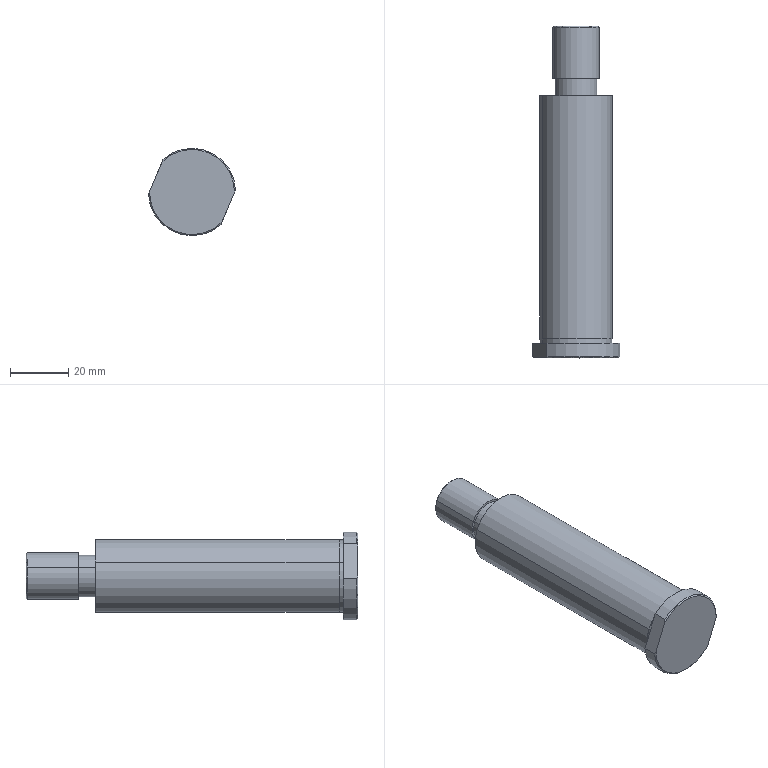Component | SolidWorks | ShaftDiameterToleranceOptionalTypeBHingePin[KPVHBH25-85]-1 | 1 solid | 22 faces | box 29.95 x 114 x 30 mm | volume 49702 mm3 | cylinder 10 | plane 8 | cone 4 | commonest cylinder face diameters 16 x2 14.4 x2 25 x2 24.8 x2 30 x2
STEP:
#1=CARTESIAN_POINT('',(4.981,-6.488,23.736));
#2=VERTEX_POINT('',#1);
#3=CARTESIAN_POINT('',(5.534,-6.488,23.508));
#4=VERTEX_POINT('',#3);
#5=CARTESIAN_POINT('',(5.257,-6.488,23.622));
#6=DIRECTION('',(-0.,1.,-0.));
#7=DIRECTION('',(0.9242,0.,-0.3818));
#8=AXIS2_PLACEMENT_3D('',#5,#6,#7);
#9=CIRCLE('',#8,0.2992);
#10=EDGE_CURVE('',#2,#4,#9,.T.);
#11=ORIENTED_EDGE('',*,*,#10,.F.);
#12=CARTESIAN_POINT('',(4.966,-6.504,23.742));
#13=VERTEX_POINT('',#12);
#14=CARTESIAN_POINT('',(4.966,-6.504,23.742));
#15=DIRECTION('',(-0.6535,-0.7071,0.27));
#16=VECTOR('',#15,39.37);
#17=LINE('',#14,#16);
#18=EDGE_CURVE('',#2,#13,#17,.T.);
#19=ORIENTED_EDGE('',*,*,#18,.T.);
#20=CARTESIAN_POINT('',(5.548,-6.504,23.502));
#21=VERTEX_POINT('',#20);
#22=CARTESIAN_POINT('',(5.257,-6.504,23.622));
#23=DIRECTION('',(0.,-1.,0.));
#24=DIRECTION('',(0.9242,0.,-0.3818));
#25=AXIS2_PLACEMENT_3D('',#22,#23,#24);
#26=CIRCLE('',#25,0.315);
#27=EDGE_CURVE('',#21,#13,#26,.T.);
#28=ORIENTED_EDGE('',*,*,#27,.F.);
#29=CARTESIAN_POINT('',(5.548,-6.504,23.502));
#30=DIRECTION('',(0.6535,-0.7071,-0.27));
#31=VECTOR('',#30,39.37);
#32=LINE('',#29,#31);
#33=EDGE_CURVE('',#4,#21,#32,.T.);
#34=ORIENTED_EDGE('',*,*,#33,.F.);
#35=EDGE_LOOP('',(#11,#19,#28,#34));
#36=FACE_OUTER_BOUND('',#35,.T.);
#37=CARTESIAN_POINT('',(5.257,-6.504,23.622));
#38=DIRECTION('',(0.,-1.,0.));
#39=DIRECTION('',(0.9242,0.,-0.3818));
#40=AXIS2_PLACEMENT_3D('',#37,#38,#39);
#41=CONICAL_SURFACE('',#40,0.315,0.7854);
#42=ADVANCED_FACE('',(#36),#41,.T.);
#43=ORIENTED_EDGE('',*,*,#27,.T.);
#44=CARTESIAN_POINT('',(4.966,-7.196,23.742));
#45=VERTEX_POINT('',#44);
#46=CARTESIAN_POINT('',(4.966,-10.976,23.742));
#47=DIRECTION('',(0.,-1.,0.));
#48=VECTOR('',#47,39.37);
#49=LINE('',#46,#48);
#50=EDGE_CURVE('',#13,#45,#49,.T.);
#51=ORIENTED_EDGE('',*,*,#50,.T.);
#52=CARTESIAN_POINT('',(5.548,-7.196,23.502));
#53=VERTEX_POINT('',#52);
#54=CARTESIAN_POINT('',(5.257,-7.196,23.622));
#55=DIRECTION('',(0.,-1.,0.));
#56=DIRECTION('',(0.9242,0.,-0.3818));
#57=AXIS2_PLACEMENT_3D('',#54,#55,#56);
#58=CIRCLE('',#57,0.315);
#59=EDGE_CURVE('',#53,#45,#58,.T.);
#60=ORIENTED_EDGE('',*,*,#59,.F.);
#61=CARTESIAN_POINT('',(5.548,-10.976,23.502));
#62=DIRECTION('',(0.,-1.,0.));
#63=VECTOR('',#62,39.37);
#64=LINE('',#61,#63);
#65=EDGE_CURVE('',#21,#53,#64,.T.);
#66=ORIENTED_EDGE('',*,*,#65,.F.);
#67=EDGE_LOOP('',(#43,#51,#60,#66));
#68=FACE_OUTER_BOUND('',#67,.T.);
#69=CARTESIAN_POINT('',(5.257,-10.976,23.622));
#70=DIRECTION('',(0.,-1.,0.));
#71=DIRECTION('',(0.9242,0.,-0.3818));
#72=AXIS2_PLACEMENT_3D('',#69,#70,#71);
#73=CYLINDRICAL_SURFACE('',#72,0.315);
#74=ADVANCED_FACE('',(#68),#73,.T.);
#75=CARTESIAN_POINT('',(5.519,-7.196,23.514));
#76=VERTEX_POINT('',#75);
#77=CARTESIAN_POINT('',(4.995,-7.196,23.73));
#78=VERTEX_POINT('',#77);
#79=CARTESIAN_POINT('',(5.257,-7.196,23.622));
#80=DIRECTION('',(0.,-1.,0.));
#81=DIRECTION('',(0.9242,0.,-0.3818));
#82=AXIS2_PLACEMENT_3D('',#79,#80,#81);
#83=CIRCLE('',#82,0.2835);
#84=EDGE_CURVE('',#76,#78,#83,.T.);
#85=ORIENTED_EDGE('',*,*,#84,.T.);
#86=CARTESIAN_POINT('',(4.995,-7.433,23.73));
#87=VERTEX_POINT('',#86);
#88=CARTESIAN_POINT('',(4.995,-10.976,23.73));
#89=DIRECTION('',(0.,-1.,0.));
#90=VECTOR('',#89,39.37);
#91=LINE('',#88,#90);
#92=EDGE_CURVE('',#78,#87,#91,.T.);
#93=ORIENTED_EDGE('',*,*,#92,.T.);
#94=CARTESIAN_POINT('',(5.519,-7.433,23.514));
#95=VERTEX_POINT('',#94);
#96=CARTESIAN_POINT('',(5.257,-7.433,23.622));
#97=DIRECTION('',(0.,-1.,0.));
#98=DIRECTION('',(0.9242,0.,-0.3818));
#99=AXIS2_PLACEMENT_3D('',#96,#97,#98);
#100=CIRCLE('',#99,0.2835);
#101=EDGE_CURVE('',#95,#87,#100,.T.);
#102=ORIENTED_EDGE('',*,*,#101,.F.);
#103=CARTESIAN_POINT('',(5.519,-10.976,23.514));
#104=DIRECTION('',(0.,-1.,0.));
#105=VECTOR('',#104,39.37);
#106=LINE('',#103,#105);
#107=EDGE_CURVE('',#76,#95,#106,.T.);
#108=ORIENTED_EDGE('',*,*,#107,.F.);
#109=EDGE_LOOP('',(#85,#93,#102,#108));
#110=FACE_OUTER_BOUND('',#109,.T.);
#111=CARTESIAN_POINT('',(5.257,-10.976,23.622));
#112=DIRECTION('',(0.,-1.,0.));
#113=DIRECTION('',(0.9242,0.,-0.3818));
#114=AXIS2_PLACEMENT_3D('',#111,#112,#113);
#115=CYLINDRICAL_SURFACE('',#114,0.2835);
#116=ADVANCED_FACE('',(#110),#115,.T.);
#117=CARTESIAN_POINT('',(5.712,-7.433,23.434));
#118=VERTEX_POINT('',#117);
#119=CARTESIAN_POINT('',(4.802,-7.433,23.81));
#120=VERTEX_POINT('',#119);
#121=CARTESIAN_POINT('',(5.257,-7.433,23.622));
#122=DIRECTION('',(0.,-1.,0.));
#123=DIRECTION('',(0.9242,0.,-0.3818));
#124=AXIS2_PLACEMENT_3D('',#121,#122,#123);
#125=CIRCLE('',#124,0.4921);
#126=EDGE_CURVE('',#118,#120,#125,.T.);
#127=ORIENTED_EDGE('',*,*,#126,.T.);
#128=CARTESIAN_POINT('',(4.802,-10.72,23.81));
#129=VERTEX_POINT('',#128);
#130=CARTESIAN_POINT('',(4.802,-10.976,23.81));
#131=DIRECTION('',(0.,-1.,0.));
#132=VECTOR('',#131,39.37);
#133=LINE('',#130,#132);
#134=EDGE_CURVE('',#120,#129,#133,.T.);
#135=ORIENTED_EDGE('',*,*,#134,.T.);
#136=CARTESIAN_POINT('',(5.712,-10.72,23.434));
#137=VERTEX_POINT('',#136);
#138=CARTESIAN_POINT('',(5.257,-10.72,23.622));
#139=DIRECTION('',(0.,-1.,0.));
#140=DIRECTION('',(0.9242,0.,-0.3818));
#141=AXIS2_PLACEMENT_3D('',#138,#139,#140);
#142=CIRCLE('',#141,0.4921);
#143=EDGE_CURVE('',#137,#129,#142,.T.);
#144=ORIENTED_EDGE('',*,*,#143,.F.);
#145=CARTESIAN_POINT('',(5.712,-10.976,23.434));
#146=DIRECTION('',(0.,-1.,0.));
#147=VECTOR('',#146,39.37);
#148=LINE('',#145,#147);
#149=EDGE_CURVE('',#118,#137,#148,.T.);
#150=ORIENTED_EDGE('',*,*,#149,.F.);
#151=EDGE_LOOP('',(#127,#135,#144,#150));
#152=FACE_OUTER_BOUND('',#151,.T.);
#153=CARTESIAN_POINT('',(5.257,-10.976,23.622));
#154=DIRECTION('',(0.,-1.,0.));
#155=DIRECTION('',(0.9242,0.,-0.3818));
#156=AXIS2_PLACEMENT_3D('',#153,#154,#155);
#157=CYLINDRICAL_SURFACE('',#156,0.4921);
#158=ADVANCED_FACE('',(#152),#157,.T.);
#159=CARTESIAN_POINT('',(5.708,-10.72,23.436));
#160=VERTEX_POINT('',#159);
#161=CARTESIAN_POINT('',(4.806,-10.72,23.808));
#162=VERTEX_POINT('',#161);
#163=CARTESIAN_POINT('',(5.257,-10.72,23.622));
#164=DIRECTION('',(0.,-1.,0.));
#165=DIRECTION('',(0.9242,0.,-0.3818));
#166=AXIS2_PLACEMENT_3D('',#163,#164,#165);
#167=CIRCLE('',#166,0.4882);
#168=EDGE_CURVE('',#160,#162,#167,.T.);
#169=ORIENTED_EDGE('',*,*,#168,.T.);
#170=CARTESIAN_POINT('',(4.806,-10.779,23.808));
#171=VERTEX_POINT('',#170);
#172=CARTESIAN_POINT('',(4.806,-10.976,23.808));
#173=DIRECTION('',(0.,-1.,0.));
#174=VECTOR('',#173,39.37);
#175=LINE('',#172,#174);
#176=EDGE_CURVE('',#162,#171,#175,.T.);
#177=ORIENTED_EDGE('',*,*,#176,.T.);
#178=CARTESIAN_POINT('',(5.708,-10.779,23.436));
#179=VERTEX_POINT('',#178);
#180=CARTESIAN_POINT('',(5.257,-10.779,23.622));
#181=DIRECTION('',(0.,-1.,0.));
#182=DIRECTION('',(0.9242,0.,-0.3818));
#183=AXIS2_PLACEMENT_3D('',#180,#181,#182);
#184=CIRCLE('',#183,0.4882);
#185=EDGE_CURVE('',#179,#171,#184,.T.);
#186=ORIENTED_EDGE('',*,*,#185,.F.);
#187=CARTESIAN_POINT('',(5.708,-10.976,23.436));
#188=DIRECTION('',(0.,-1.,0.));
#189=VECTOR('',#188,39.37);
#190=LINE('',#187,#189);
#191=EDGE_CURVE('',#160,#179,#190,.T.);
#192=ORIENTED_EDGE('',*,*,#191,.F.);
#193=EDGE_LOOP('',(#169,#177,#186,#192));
#194=FACE_OUTER_BOUND('',#193,.T.);
#195=CARTESIAN_POINT('',(5.257,-10.976,23.622));
#196=DIRECTION('',(0.,-1.,0.));
#197=DIRECTION('',(0.9242,0.,-0.3818));
#198=AXIS2_PLACEMENT_3D('',#195,#196,#197);
#199=CYLINDRICAL_SURFACE('',#198,0.4882);
#200=ADVANCED_FACE('',(#194),#199,.T.);
#201=CARTESIAN_POINT('',(5.65,-10.779,23.181));
#202=VERTEX_POINT('',#201);
#203=CARTESIAN_POINT('',(5.65,-10.96,23.181));
#204=VERTEX_POINT('',#203);
#205=CARTESIAN_POINT('',(5.65,-10.779,23.181));
#206=DIRECTION('',(0.,-1.,0.));
#207=VECTOR('',#206,39.37);
#208=LINE('',#205,#207);
#209=EDGE_CURVE('',#202,#204,#208,.T.);
#210=ORIENTED_EDGE('',*,*,#209,.T.);
#211=CARTESIAN_POINT('',(4.668,-10.96,23.587));
#212=VERTEX_POINT('',#211);
#213=CARTESIAN_POINT('',(5.257,-10.96,23.622));
#214=DIRECTION('',(-0.,1.,-0.));
#215=DIRECTION('',(-0.9242,-0.,0.3818));
#216=AXIS2_PLACEMENT_3D('',#213,#214,#215);
#217=CIRCLE('',#216,0.5906);
#218=EDGE_CURVE('',#204,#212,#217,.T.);
#219=ORIENTED_EDGE('',*,*,#218,.T.);
#220=CARTESIAN_POINT('',(4.668,-10.779,23.587));
#221=VERTEX_POINT('',#220);
#222=CARTESIAN_POINT('',(4.668,-10.779,23.587));
#223=DIRECTION('',(0.,-1.,0.));
#224=VECTOR('',#223,39.37);
#225=LINE('',#222,#224);
#226=EDGE_CURVE('',#221,#212,#225,.T.);
#227=ORIENTED_EDGE('',*,*,#226,.F.);
#228=CARTESIAN_POINT('',(5.257,-10.779,23.622));
#229=DIRECTION('',(0.,-1.,0.));
#230=DIRECTION('',(0.9242,0.,-0.3818));
#231=AXIS2_PLACEMENT_3D('',#228,#229,#230);
#232=CIRCLE('',#231,0.5906);
#233=EDGE_CURVE('',#221,#202,#232,.T.);
#234=ORIENTED_EDGE('',*,*,#233,.T.);
#235=EDGE_LOOP('',(#210,#219,#227,#234));
#236=FACE_OUTER_BOUND('',#235,.T.);
#237=CARTESIAN_POINT('',(5.257,-10.976,23.622));
#238=DIRECTION('',(0.,-1.,0.));
#239=DIRECTION('',(0.9242,0.,-0.3818));
#240=AXIS2_PLACEMENT_3D('',#237,#238,#239);
#241=CYLINDRICAL_SURFACE('',#240,0.5906);
#242=ADVANCED_FACE('',(#236),#241,.T.);
#243=CARTESIAN_POINT('',(4.864,-10.779,24.063));
#244=VERTEX_POINT('',#243);
#245=CARTESIAN_POINT('',(4.864,-10.96,24.063));
#246=VERTEX_POINT('',#245);
#247=CARTESIAN_POINT('',(4.864,-10.779,24.063));
#248=DIRECTION('',(0.,-1.,0.));
#249=VECTOR('',#248,39.37);
#250=LINE('',#247,#249);
#251=EDGE_CURVE('',#244,#246,#250,.T.);
#252=ORIENTED_EDGE('',*,*,#251,.T.);
#253=CARTESIAN_POINT('',(5.847,-10.96,23.657));
#254=VERTEX_POINT('',#253);
#255=CARTESIAN_POINT('',(5.257,-10.96,23.622));
#256=DIRECTION('',(-0.,1.,-0.));
#257=DIRECTION('',(-0.9242,-0.,0.3818));
#258=AXIS2_PLACEMENT_3D('',#255,#256,#257);
#259=CIRCLE('',#258,0.5906);
#260=EDGE_CURVE('',#246,#254,#259,.T.);
#261=ORIENTED_EDGE('',*,*,#260,.T.);
#262=CARTESIAN_POINT('',(5.847,-10.779,23.657));
#263=VERTEX_POINT('',#262);
#264=CARTESIAN_POINT('',(5.847,-10.779,23.657));
#265=DIRECTION('',(0.,-1.,0.));
#266=VECTOR('',#265,39.37);
#267=LINE('',#264,#266);
#268=EDGE_CURVE('',#263,#254,#267,.T.);
#269=ORIENTED_EDGE('',*,*,#268,.F.);
#270=CARTESIAN_POINT('',(5.257,-10.779,23.622));
#271=DIRECTION('',(0.,-1.,0.));
#272=DIRECTION('',(0.9242,0.,-0.3818));
#273=AXIS2_PLACEMENT_3D('',#270,#271,#272);
#274=CIRCLE('',#273,0.5906);
#275=EDGE_CURVE('',#263,#244,#274,.T.);
#276=ORIENTED_EDGE('',*,*,#275,.T.);
#277=EDGE_LOOP('',(#252,#261,#269,#276));
#278=FACE_OUTER_BOUND('',#277,.T.);
#279=CARTESIAN_POINT('',(5.257,-10.976,23.622));
#280=DIRECTION('',(0.,-1.,0.));
#281=DIRECTION('',(0.9242,0.,-0.3818));
#282=AXIS2_PLACEMENT_3D('',#279,#280,#281);
#283=CYLINDRICAL_SURFACE('',#282,0.5906);
#284=ADVANCED_FACE('',(#278),#283,.T.);
#285=ORIENTED_EDGE('',*,*,#275,.F.);
#286=CARTESIAN_POINT('',(5.847,-10.779,23.657));
#287=DIRECTION('',(-0.3818,-0.,-0.9242));
#288=VECTOR('',#287,39.37);
#289=LINE('',#286,#288);
#290=EDGE_CURVE('',#263,#202,#289,.T.);
#291=ORIENTED_EDGE('',*,*,#290,.T.);
#292=ORIENTED_EDGE('',*,*,#233,.F.);
#293=CARTESIAN_POINT('',(4.864,-10.779,24.063));
#294=DIRECTION('',(0.3818,0.,0.9242));
#295=VECTOR('',#294,39.37);
#296=LINE('',#293,#295);
#297=EDGE_CURVE('',#221,#244,#296,.T.);
#298=ORIENTED_EDGE('',*,*,#297,.T.);
#299=EDGE_LOOP('',(#285,#291,#292,#298));
#300=FACE_OUTER_BOUND('',#299,.T.);
#301=ORIENTED_EDGE('',*,*,#185,.T.);
#302=CARTESIAN_POINT('',(5.257,-10.779,23.622));
#303=DIRECTION('',(0.,-1.,0.));
#304=DIRECTION('',(0.9242,0.,-0.3818));
#305=AXIS2_PLACEMENT_3D('',#302,#303,#304);
#306=CIRCLE('',#305,0.4882);
#307=EDGE_CURVE('',#171,#179,#306,.T.);
#308=ORIENTED_EDGE('',*,*,#307,.T.);
#309=EDGE_LOOP('',(#301,#308));
#310=FACE_BOUND('',#309,.T.);
#311=CARTESIAN_POINT('',(5.483,-10.779,24.168));
#312=DIRECTION('',(0.,-1.,0.));
#313=DIRECTION('',(0.9242,0.,-0.3818));
#314=AXIS2_PLACEMENT_3D('',#311,#312,#313);
#315=PLANE('',#314);
#316=ADVANCED_FACE('',(#300,#310),#315,.F.);
#317=ORIENTED_EDGE('',*,*,#176,.F.);
#318=CARTESIAN_POINT('',(5.257,-10.72,23.622));
#319=DIRECTION('',(0.,-1.,0.));
#320=DIRECTION('',(0.9242,0.,-0.3818));
#321=AXIS2_PLACEMENT_3D('',#318,#319,#320);
#322=CIRCLE('',#321,0.4882);
#323=EDGE_CURVE('',#162,#160,#322,.T.);
#324=ORIENTED_EDGE('',*,*,#323,.T.);
#325=ORIENTED_EDGE('',*,*,#191,.T.);
#326=ORIENTED_EDGE('',*,*,#307,.F.);
#327=EDGE_LOOP('',(#317,#324,#325,#326));
#328=FACE_OUTER_BOUND('',#327,.T.);
#329=CARTESIAN_POINT('',(5.257,-10.976,23.622));
#330=DIRECTION('',(0.,-1.,0.));
#331=DIRECTION('',(0.9242,0.,-0.3818));
#332=AXIS2_PLACEMENT_3D('',#329,#330,#331);
#333=CYLINDRICAL_SURFACE('',#332,0.4882);
#334=ADVANCED_FACE('',(#328),#333,.T.);
#335=ORIENTED_EDGE('',*,*,#168,.F.);
#336=ORIENTED_EDGE('',*,*,#323,.F.);
#337=EDGE_LOOP('',(#335,#336));
#338=FACE_BOUND('',#337,.T.);
#339=ORIENTED_EDGE('',*,*,#143,.T.);
#340=CARTESIAN_POINT('',(5.257,-10.72,23.622));
#341=DIRECTION('',(0.,-1.,0.));
#342=DIRECTION('',(0.9242,0.,-0.3818));
#343=AXIS2_PLACEMENT_3D('',#340,#341,#342);
#344=CIRCLE('',#343,0.4921);
#345=EDGE_CURVE('',#129,#137,#344,.T.);
#346=ORIENTED_EDGE('',*,*,#345,.T.);
#347=EDGE_LOOP('',(#339,#346));
#348=FACE_OUTER_BOUND('',#347,.T.);
#349=CARTESIAN_POINT('',(5.443,-10.72,24.073));
#350=DIRECTION('',(-0.,1.,-0.));
#351=DIRECTION('',(-0.9242,-0.,0.3818));
#352=AXIS2_PLACEMENT_3D('',#349,#350,#351);
#353=PLANE('',#352);
#354=ADVANCED_FACE('',(#338,#348),#353,.F.);
#355=ORIENTED_EDGE('',*,*,#134,.F.);
#356=CARTESIAN_POINT('',(5.257,-7.433,23.622));
#357=DIRECTION('',(0.,-1.,0.));
#358=DIRECTION('',(0.9242,0.,-0.3818));
#359=AXIS2_PLACEMENT_3D('',#356,#357,#358);
#360=CIRCLE('',#359,0.4921);
#361=EDGE_CURVE('',#120,#118,#360,.T.);
#362=ORIENTED_EDGE('',*,*,#361,.T.);
#363=ORIENTED_EDGE('',*,*,#149,.T.);
#364=ORIENTED_EDGE('',*,*,#345,.F.);
#365=EDGE_LOOP('',(#355,#362,#363,#364));
#366=FACE_OUTER_BOUND('',#365,.T.);
#367=CARTESIAN_POINT('',(5.257,-10.976,23.622));
#368=DIRECTION('',(0.,-1.,0.));
#369=DIRECTION('',(0.9242,0.,-0.3818));
#370=AXIS2_PLACEMENT_3D('',#367,#368,#369);
#371=CYLINDRICAL_SURFACE('',#370,0.4921);
#372=ADVANCED_FACE('',(#366),#371,.T.);
#373=ORIENTED_EDGE('',*,*,#126,.F.);
#374=ORIENTED_EDGE('',*,*,#361,.F.);
#375=EDGE_LOOP('',(#373,#374));
#376=FACE_OUTER_BOUND('',#375,.T.);
#377=ORIENTED_EDGE('',*,*,#101,.T.);
#378=CARTESIAN_POINT('',(5.257,-7.433,23.622));
#379=DIRECTION('',(0.,-1.,0.));
#380=DIRECTION('',(0.9242,0.,-0.3818));
#381=AXIS2_PLACEMENT_3D('',#378,#379,#380);
#382=CIRCLE('',#381,0.2835);
#383=EDGE_CURVE('',#87,#95,#382,.T.);
#384=ORIENTED_EDGE('',*,*,#383,.T.);
#385=EDGE_LOOP('',(#377,#384));
#386=FACE_BOUND('',#385,.T.);
#387=CARTESIAN_POINT('',(5.445,-7.433,24.077));
#388=DIRECTION('',(0.,-1.,0.));
#389=DIRECTION('',(0.9242,0.,-0.3818));
#390=AXIS2_PLACEMENT_3D('',#387,#388,#389);
#391=PLANE('',#390);
#392=ADVANCED_FACE('',(#376,#386),#391,.F.);
#393=ORIENTED_EDGE('',*,*,#92,.F.);
#394=CARTESIAN_POINT('',(5.257,-7.196,23.622));
#395=DIRECTION('',(0.,-1.,0.));
#396=DIRECTION('',(0.9242,0.,-0.3818));
#397=AXIS2_PLACEMENT_3D('',#394,#395,#396);
#398=CIRCLE('',#397,0.2835);
#399=EDGE_CURVE('',#78,#76,#398,.T.);
#400=ORIENTED_EDGE('',*,*,#399,.T.);
#401=ORIENTED_EDGE('',*,*,#107,.T.);
#402=ORIENTED_EDGE('',*,*,#383,.F.);
#403=EDGE_LOOP('',(#393,#400,#401,#402));
#404=FACE_OUTER_BOUND('',#403,.T.);
#405=CARTESIAN_POINT('',(5.257,-10.976,23.622));
#406=DIRECTION('',(0.,-1.,0.));
#407=DIRECTION('',(0.9242,0.,-0.3818));
#408=AXIS2_PLACEMENT_3D('',#405,#406,#407);
#409=CYLINDRICAL_SURFACE('',#408,0.2835);
#410=ADVANCED_FACE('',(#404),#409,.T.);
#411=ORIENTED_EDGE('',*,*,#84,.F.);
#412=ORIENTED_EDGE('',*,*,#399,.F.);
#413=EDGE_LOOP('',(#411,#412));
#414=FACE_BOUND('',#413,.T.);
#415=ORIENTED_EDGE('',*,*,#59,.T.);
#416=CARTESIAN_POINT('',(5.257,-7.196,23.622));
#417=DIRECTION('',(0.,-1.,0.));
#418=DIRECTION('',(0.9242,0.,-0.3818));
#419=AXIS2_PLACEMENT_3D('',#416,#417,#418);
#420=CIRCLE('',#419,0.315);
#421=EDGE_CURVE('',#45,#53,#420,.T.);
#422=ORIENTED_EDGE('',*,*,#421,.T.);
#423=EDGE_LOOP('',(#415,#422));
#424=FACE_OUTER_BOUND('',#423,.T.);
#425=CARTESIAN_POINT('',(5.365,-7.196,23.884));
#426=DIRECTION('',(-0.,1.,-0.));
#427=DIRECTION('',(-0.9242,-0.,0.3818));
#428=AXIS2_PLACEMENT_3D('',#425,#426,#427);
#429=PLANE('',#428);
#430=ADVANCED_FACE('',(#414,#424),#429,.F.);
#431=ORIENTED_EDGE('',*,*,#50,.F.);
#432=CARTESIAN_POINT('',(5.257,-6.504,23.622));
#433=DIRECTION('',(0.,-1.,0.));
#434=DIRECTION('',(0.9242,0.,-0.3818));
#435=AXIS2_PLACEMENT_3D('',#432,#433,#434);
#436=CIRCLE('',#435,0.315);
#437=EDGE_CURVE('',#13,#21,#436,.T.);
#438=ORIENTED_EDGE('',*,*,#437,.T.);
#439=ORIENTED_EDGE('',*,*,#65,.T.);
#440=ORIENTED_EDGE('',*,*,#421,.F.);
#441=EDGE_LOOP('',(#431,#438,#439,#440));
#442=FACE_OUTER_BOUND('',#441,.T.);
#443=CARTESIAN_POINT('',(5.257,-10.976,23.622));
#444=DIRECTION('',(0.,-1.,0.));
#445=DIRECTION('',(0.9242,0.,-0.3818));
#446=AXIS2_PLACEMENT_3D('',#443,#444,#445);
#447=CYLINDRICAL_SURFACE('',#446,0.315);
#448=ADVANCED_FACE('',(#442),#447,.T.);
#449=CARTESIAN_POINT('',(5.257,-6.488,23.622));
#450=DIRECTION('',(-0.,1.,-0.));
#451=DIRECTION('',(0.9242,0.,-0.3818));
#452=AXIS2_PLACEMENT_3D('',#449,#450,#451);
#453=CIRCLE('',#452,0.2992);
#454=EDGE_CURVE('',#4,#2,#453,.T.);
#455=ORIENTED_EDGE('',*,*,#454,.T.);
#456=ORIENTED_EDGE('',*,*,#10,.T.);
#457=EDGE_LOOP('',(#455,#456));
#458=FACE_OUTER_BOUND('',#457,.T.);
#459=CARTESIAN_POINT('',(5.377,-6.488,23.913));
#460=DIRECTION('',(0.,-1.,0.));
#461=DIRECTION('',(0.9242,0.,-0.3818));
#462=AXIS2_PLACEMENT_3D('',#459,#460,#461);
#463=PLANE('',#462);
#464=ADVANCED_FACE('',(#458),#463,.F.);
#465=CARTESIAN_POINT('',(4.682,-10.976,23.623));
#466=VERTEX_POINT('',#465);
#467=CARTESIAN_POINT('',(4.849,-10.976,24.027));
#468=VERTEX_POINT('',#467);
#469=CARTESIAN_POINT('',(4.864,-10.976,24.063));
#470=DIRECTION('',(0.3818,0.,0.9242));
#471=VECTOR('',#470,39.37);
#472=LINE('',#469,#471);
#473=EDGE_CURVE('',#466,#468,#472,.T.);
#474=ORIENTED_EDGE('',*,*,#473,.F.);
#475=CARTESIAN_POINT('',(5.665,-10.976,23.217));
#476=VERTEX_POINT('',#475);
#477=CARTESIAN_POINT('',(5.257,-10.976,23.622));
#478=DIRECTION('',(0.,-1.,0.));
#479=DIRECTION('',(-0.9242,-0.,0.3818));
#480=AXIS2_PLACEMENT_3D('',#477,#478,#479);
#481=CIRCLE('',#480,0.5748);
#482=EDGE_CURVE('',#466,#476,#481,.T.);
#483=ORIENTED_EDGE('',*,*,#482,.T.);
#484=CARTESIAN_POINT('',(5.832,-10.976,23.621));
#485=VERTEX_POINT('',#484);
#486=CARTESIAN_POINT('',(5.847,-10.976,23.657));
#487=DIRECTION('',(-0.3818,-0.,-0.9242));
#488=VECTOR('',#487,39.37);
#489=LINE('',#486,#488);
#490=EDGE_CURVE('',#485,#476,#489,.T.);
#491=ORIENTED_EDGE('',*,*,#490,.F.);
#492=CARTESIAN_POINT('',(5.257,-10.976,23.622));
#493=DIRECTION('',(0.,-1.,0.));
#494=DIRECTION('',(-0.9242,-0.,0.3818));
#495=AXIS2_PLACEMENT_3D('',#492,#493,#494);
#496=CIRCLE('',#495,0.5748);
#497=EDGE_CURVE('',#485,#468,#496,.T.);
#498=ORIENTED_EDGE('',*,*,#497,.T.);
#499=EDGE_LOOP('',(#474,#483,#491,#498));
#500=FACE_OUTER_BOUND('',#499,.T.);
#501=CARTESIAN_POINT('',(5.483,-10.976,24.168));
#502=DIRECTION('',(-0.,1.,-0.));
#503=DIRECTION('',(-0.9242,-0.,0.3818));
#504=AXIS2_PLACEMENT_3D('',#501,#502,#503);
#505=PLANE('',#504);
#506=ADVANCED_FACE('',(#500),#505,.F.);
#507=ORIENTED_EDGE('',*,*,#226,.T.);
#508=CARTESIAN_POINT('',(4.668,-10.96,23.587));
#509=CARTESIAN_POINT('',(4.672,-10.966,23.599));
#510=CARTESIAN_POINT('',(4.677,-10.971,23.611));
#511=CARTESIAN_POINT('',(4.682,-10.976,23.623));
#512=B_SPLINE_CURVE_WITH_KNOTS('',3,(#508,#509,#510,#511),.UNSPECIFIED.,.F.,.F.,(4,4),(0.,0.001057),.UNSPECIFIED.);
#513=EDGE_CURVE('',#212,#466,#512,.T.);
#514=ORIENTED_EDGE('',*,*,#513,.T.);
#515=ORIENTED_EDGE('',*,*,#473,.T.);
#516=CARTESIAN_POINT('',(4.849,-10.976,24.027));
#517=CARTESIAN_POINT('',(4.854,-10.971,24.039));
#518=CARTESIAN_POINT('',(4.859,-10.966,24.051));
#519=CARTESIAN_POINT('',(4.864,-10.96,24.063));
#520=B_SPLINE_CURVE_WITH_KNOTS('',3,(#516,#517,#518,#519),.UNSPECIFIED.,.F.,.F.,(4,4),(0.,0.001057),.UNSPECIFIED.);
#521=EDGE_CURVE('',#468,#246,#520,.T.);
#522=ORIENTED_EDGE('',*,*,#521,.T.);
#523=ORIENTED_EDGE('',*,*,#251,.F.);
#524=ORIENTED_EDGE('',*,*,#297,.F.);
#525=EDGE_LOOP('',(#507,#514,#515,#522,#523,#524));
#526=FACE_OUTER_BOUND('',#525,.T.);
#527=CARTESIAN_POINT('',(4.864,-10.779,24.063));
#528=DIRECTION('',(0.9242,0.,-0.3818));
#529=DIRECTION('',(-0.,1.,-0.));
#530=AXIS2_PLACEMENT_3D('',#527,#528,#529);
#531=PLANE('',#530);
#532=ADVANCED_FACE('',(#526),#531,.F.);
#533=ORIENTED_EDGE('',*,*,#490,.T.);
#534=CARTESIAN_POINT('',(5.665,-10.976,23.217));
#535=CARTESIAN_POINT('',(5.66,-10.971,23.205));
#536=CARTESIAN_POINT('',(5.655,-10.966,23.193));
#537=CARTESIAN_POINT('',(5.65,-10.96,23.181));
#538=B_SPLINE_CURVE_WITH_KNOTS('',3,(#534,#535,#536,#537),.UNSPECIFIED.,.F.,.F.,(4,4),(0.,0.001057),.UNSPECIFIED.);
#539=EDGE_CURVE('',#476,#204,#538,.T.);
#540=ORIENTED_EDGE('',*,*,#539,.T.);
#541=ORIENTED_EDGE('',*,*,#209,.F.);
#542=ORIENTED_EDGE('',*,*,#290,.F.);
#543=ORIENTED_EDGE('',*,*,#268,.T.);
#544=CARTESIAN_POINT('',(5.847,-10.96,23.657));
#545=CARTESIAN_POINT('',(5.842,-10.966,23.645));
#546=CARTESIAN_POINT('',(5.837,-10.971,23.633));
#547=CARTESIAN_POINT('',(5.832,-10.976,23.621));
#548=B_SPLINE_CURVE_WITH_KNOTS('',3,(#544,#545,#546,#547),.UNSPECIFIED.,.F.,.F.,(4,4),(0.,0.001057),.UNSPECIFIED.);
#549=EDGE_CURVE('',#254,#485,#548,.T.);
#550=ORIENTED_EDGE('',*,*,#549,.T.);
#551=EDGE_LOOP('',(#533,#540,#541,#542,#543,#550));
#552=FACE_OUTER_BOUND('',#551,.T.);
#553=CARTESIAN_POINT('',(5.847,-10.779,23.657));
#554=DIRECTION('',(-0.9242,-0.,0.3818));
#555=DIRECTION('',(0.,-1.,0.));
#556=AXIS2_PLACEMENT_3D('',#553,#554,#555);
#557=PLANE('',#556);
#558=ADVANCED_FACE('',(#552),#557,.F.);
#559=ORIENTED_EDGE('',*,*,#18,.F.);
#560=ORIENTED_EDGE('',*,*,#454,.F.);
#561=ORIENTED_EDGE('',*,*,#33,.T.);
#562=ORIENTED_EDGE('',*,*,#437,.F.);
#563=EDGE_LOOP('',(#559,#560,#561,#562));
#564=FACE_OUTER_BOUND('',#563,.T.);
#565=CARTESIAN_POINT('',(5.257,-6.504,23.622));
#566=DIRECTION('',(0.,-1.,0.));
#567=DIRECTION('',(0.9242,0.,-0.3818));
#568=AXIS2_PLACEMENT_3D('',#565,#566,#567);
#569=CONICAL_SURFACE('',#568,0.315,0.7854);
#570=ADVANCED_FACE('',(#564),#569,.T.);
#571=ORIENTED_EDGE('',*,*,#513,.F.);
#572=ORIENTED_EDGE('',*,*,#218,.F.);
#573=ORIENTED_EDGE('',*,*,#539,.F.);
#574=ORIENTED_EDGE('',*,*,#482,.F.);
#575=EDGE_LOOP('',(#571,#572,#573,#574));
#576=FACE_OUTER_BOUND('',#575,.T.);
#577=CARTESIAN_POINT('',(5.257,-10.976,23.622));
#578=DIRECTION('',(-0.,1.,-0.));
#579=DIRECTION('',(-0.9242,-0.,0.3818));
#580=AXIS2_PLACEMENT_3D('',#577,#578,#579);
#581=CONICAL_SURFACE('',#580,0.5748,0.7854);
#582=ADVANCED_FACE('',(#576),#581,.T.);
#583=ORIENTED_EDGE('',*,*,#549,.F.);
#584=ORIENTED_EDGE('',*,*,#260,.F.);
#585=ORIENTED_EDGE('',*,*,#521,.F.);
#586=ORIENTED_EDGE('',*,*,#497,.F.);
#587=EDGE_LOOP('',(#583,#584,#585,#586));
#588=FACE_OUTER_BOUND('',#587,.T.);
#589=CARTESIAN_POINT('',(5.257,-10.976,23.622));
#590=DIRECTION('',(-0.,1.,-0.));
#591=DIRECTION('',(-0.9242,-0.,0.3818));
#592=AXIS2_PLACEMENT_3D('',#589,#590,#591);
#593=CONICAL_SURFACE('',#592,0.5748,0.7854);
#594=ADVANCED_FACE('',(#588),#593,.T.);
#595=CLOSED_SHELL('',(#42,#74,#116,#158,#200,#242,#284,#316,#334,#354,#372,#392,#410,#430,#448,#464,#506,#532,#558,#570,#582,#594));
#596=MANIFOLD_SOLID_BREP('',#595);
#597=CARTESIAN_POINT('',(0.,0.,0.));
#598=DIRECTION('',(0.,0.,1.));
#599=DIRECTION('',(1.,0.,0.));
#600=AXIS2_PLACEMENT_3D('',#597,#598,#599);
#601=(LENGTH_UNIT()NAMED_UNIT(*)SI_UNIT($,.METRE.));
#602=LENGTH_MEASURE_WITH_UNIT(LENGTH_MEASURE(0.0254),#601);
#603=DIMENSIONAL_EXPONENTS(1.,0.,0.,0.,0.,0.,0.);
#604=(CONVERSION_BASED_UNIT('',#602)LENGTH_UNIT()NAMED_UNIT(#603));
#605=UNCERTAINTY_MEASURE_WITH_UNIT(LENGTH_MEASURE(0.00001),#604,'','');
#606=(NAMED_UNIT(*)PLANE_ANGLE_UNIT()SI_UNIT($,.RADIAN.));
#607=(NAMED_UNIT(*)SI_UNIT($,.STERADIAN.)SOLID_ANGLE_UNIT());
#608=(GEOMETRIC_REPRESENTATION_CONTEXT(3)GLOBAL_UNCERTAINTY_ASSIGNED_CONTEXT((#605))GLOBAL_UNIT_ASSIGNED_CONTEXT((#604,#606,#607))REPRESENTATION_CONTEXT('',''));
#609=ADVANCED_BREP_SHAPE_REPRESENTATION('',(#596,#600),#608);
#610=COLOUR_RGB('',0.7922,0.8196,0.9333);
#611=FILL_AREA_STYLE_COLOUR('',#610);
#612=FILL_AREA_STYLE('',(#611));
#613=SURFACE_STYLE_FILL_AREA(#612);
#614=SURFACE_SIDE_STYLE('',(#613));
#615=SURFACE_STYLE_USAGE(.BOTH.,#614);
#616=PRESENTATION_STYLE_ASSIGNMENT((#615));
#617=STYLED_ITEM('',(#616),#596);
#618=(LENGTH_UNIT()NAMED_UNIT(*)SI_UNIT($,.METRE.));
#619=LENGTH_MEASURE_WITH_UNIT(LENGTH_MEASURE(0.0254),#618);
#620=DIMENSIONAL_EXPONENTS(1.,0.,0.,0.,0.,0.,0.);
#621=(CONVERSION_BASED_UNIT('',#619)LENGTH_UNIT()NAMED_UNIT(#620));
#622=UNCERTAINTY_MEASURE_WITH_UNIT(LENGTH_MEASURE(0.00001),#621,'','');
#623=(NAMED_UNIT(*)PLANE_ANGLE_UNIT()SI_UNIT($,.RADIAN.));
#624=(NAMED_UNIT(*)SI_UNIT($,.STERADIAN.)SOLID_ANGLE_UNIT());
#625=(GEOMETRIC_REPRESENTATION_CONTEXT(3)GLOBAL_UNCERTAINTY_ASSIGNED_CONTEXT((#622))GLOBAL_UNIT_ASSIGNED_CONTEXT((#621,#623,#624))REPRESENTATION_CONTEXT('',''));
#626=MECHANICAL_DESIGN_GEOMETRIC_PRESENTATION_REPRESENTATION('',(#617),#625);
#627=PRESENTATION_LAYER_ASSIGNMENT('','',(#617));